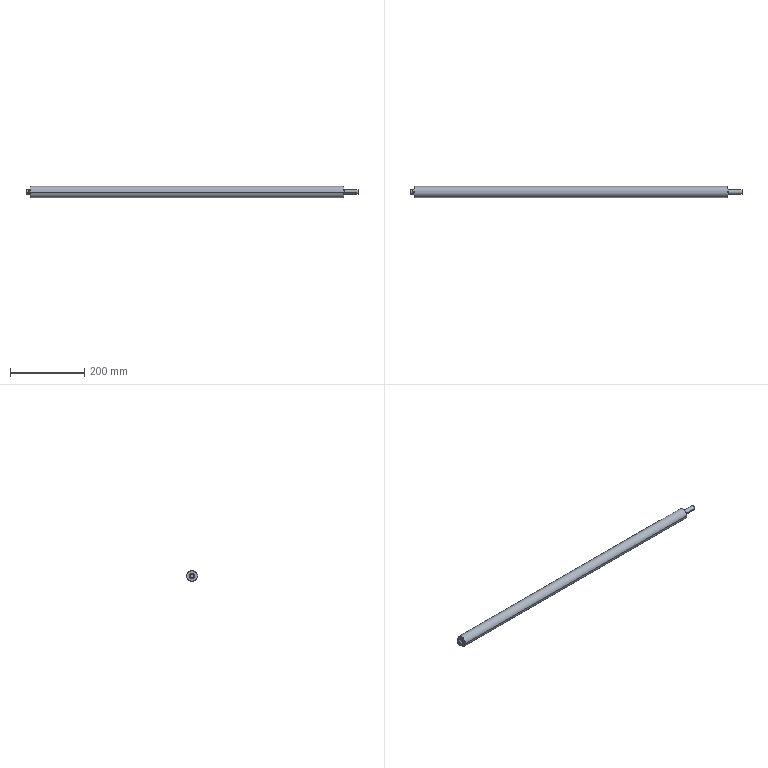Component | SolidWorks | DriveAxis-1_MainFeedAxis3-1 | 1 solid | 26 faces | box 892 x 30 x 30 mm | volume 601650 mm3 | cone 10 | cylinder 10 | plane 6 | commonest cylinder face diameters 12 x4 15 x4 30 x2
build123d program:
from build123d import *

# Parameters (mm, degrees)
SKETCH1_R           = 15
BOSS_EXTRUDE1_DEPTH = 843
SKETCH3_R           = 7.5
BOSS_EXTRUDE2_DEPTH = 3
BOSS_EXTRUDE3_START = 3
SKETCH4_R           = 7.5
BOSS_EXTRUDE3_DEPTH = 3
SKETCH5_R           = 6
BOSS_EXTRUDE4_DEPTH = 35
BOSS_EXTRUDE5_START = 8
SKETCH6_R           = 6
BOSS_EXTRUDE5_DEPTH = 8
CHAMFER1_SIZE       = 1
CHAMFER2_SIZE       = 1


with BuildPart() as part:
    # Sketch1 → Boss-Extrude1 (new body)
    with BuildSketch(Plane.XY):
        with Locations(Location((0, 0, 0), (0, 0, 180))):
            Circle(SKETCH1_R)
    extrude(amount=BOSS_EXTRUDE1_DEPTH)

    # Sketch3 → Boss-Extrude2 (add)
    with BuildSketch(Plane.XY.offset(843)):
        Circle(SKETCH3_R)
    extrude(amount=BOSS_EXTRUDE2_DEPTH)

    # Sketch4 → Boss-Extrude3 (add)
    with BuildSketch(Plane(origin=(0, 0, 0), x_dir=(-1, 0, 0), z_dir=(0, 0, -1)).offset(BOSS_EXTRUDE3_START)):
        with Locations(Location((0, 0, 0), (0, 0, 180))):
            Circle(SKETCH4_R)
    extrude(amount=-BOSS_EXTRUDE3_DEPTH)

    # Sketch5 → Boss-Extrude4 (add)
    with BuildSketch(Plane(origin=(0, 0, -3), x_dir=(-1, 0, 0), z_dir=(0, 0, -1))):
        Circle(SKETCH5_R)
    extrude(amount=BOSS_EXTRUDE4_DEPTH)

    # Sketch6 → Boss-Extrude5 (add)
    with BuildSketch(Plane.XY.offset(846).offset(BOSS_EXTRUDE5_START)):
        with Locations(Location((0, 0, 0), (0, 0, 180))):
            Circle(SKETCH6_R)
    extrude(amount=-BOSS_EXTRUDE5_DEPTH)

    # Chamfer1
    chamfer1_edges = [part.edges().sort_by_distance(p)[0] for p in [
        (6, 0, 854),
        (15, 0, 843),
        (-7.5, 0, 846),
    ]]
    chamfer(chamfer1_edges, length=CHAMFER1_SIZE)

    # Chamfer2
    chamfer2_edges = [part.edges().sort_by_distance(p)[0] for p in [
        (-7.5, 0, -3),
        (15, 0, 0),
    ]]
    chamfer(chamfer2_edges, length=CHAMFER2_SIZE)


solid = part.part

# Placed as in the assembly
solid = solid.moved(Location((856, -30, -142.268), (0, -90, 0)))
STEP:
#1=COLOUR_RGB('',0.7922,0.8196,0.9333);
#2=FILL_AREA_STYLE_COLOUR('',#1);
#3=FILL_AREA_STYLE('',(#2));
#4=SURFACE_STYLE_FILL_AREA(#3);
#5=SURFACE_SIDE_STYLE('',(#4));
#6=SURFACE_STYLE_USAGE(.BOTH.,#5);
#7=PRESENTATION_STYLE_ASSIGNMENT((#6));
#8=CARTESIAN_POINT('',(33.701,-1.732,-5.601));
#9=VERTEX_POINT('',#8);
#10=CARTESIAN_POINT('',(33.701,-0.6299,-5.601));
#11=VERTEX_POINT('',#10);
#12=CARTESIAN_POINT('',(33.701,-1.181,-5.601));
#13=DIRECTION('',(1.,0.,0.));
#14=DIRECTION('',(0.,1.,0.));
#15=AXIS2_PLACEMENT_3D('',#12,#13,#14);
#16=CIRCLE('',#15,0.5512);
#17=EDGE_CURVE('',#9,#11,#16,.T.);
#18=ORIENTED_EDGE('',*,*,#17,.F.);
#19=CARTESIAN_POINT('',(33.661,-1.772,-5.601));
#20=VERTEX_POINT('',#19);
#21=CARTESIAN_POINT('',(33.661,-1.772,-5.601));
#22=DIRECTION('',(-0.7071,-0.7071,-0.));
#23=VECTOR('',#22,39.37);
#24=LINE('',#21,#23);
#25=EDGE_CURVE('',#9,#20,#24,.T.);
#26=ORIENTED_EDGE('',*,*,#25,.T.);
#27=CARTESIAN_POINT('',(33.661,-0.5906,-5.601));
#28=VERTEX_POINT('',#27);
#29=CARTESIAN_POINT('',(33.661,-1.181,-5.601));
#30=DIRECTION('',(-1.,-0.,-0.));
#31=DIRECTION('',(0.,1.,0.));
#32=AXIS2_PLACEMENT_3D('',#29,#30,#31);
#33=CIRCLE('',#32,0.5906);
#34=EDGE_CURVE('',#28,#20,#33,.T.);
#35=ORIENTED_EDGE('',*,*,#34,.F.);
#36=CARTESIAN_POINT('',(33.661,-0.5906,-5.601));
#37=DIRECTION('',(-0.7071,0.7071,0.));
#38=VECTOR('',#37,39.37);
#39=LINE('',#36,#38);
#40=EDGE_CURVE('',#11,#28,#39,.T.);
#41=ORIENTED_EDGE('',*,*,#40,.F.);
#42=EDGE_LOOP('',(#18,#26,#35,#41));
#43=FACE_OUTER_BOUND('',#42,.T.);
#44=CARTESIAN_POINT('',(33.661,-1.181,-5.601));
#45=DIRECTION('',(-1.,-0.,-0.));
#46=DIRECTION('',(0.,1.,0.));
#47=AXIS2_PLACEMENT_3D('',#44,#45,#46);
#48=CONICAL_SURFACE('',#47,0.5906,0.7854);
#49=ADVANCED_FACE('',(#43),#48,.T.);
#50=CARTESIAN_POINT('',(33.819,-1.437,-5.601));
#51=VERTEX_POINT('',#50);
#52=CARTESIAN_POINT('',(33.819,-0.9252,-5.601));
#53=VERTEX_POINT('',#52);
#54=CARTESIAN_POINT('',(33.819,-1.181,-5.601));
#55=DIRECTION('',(1.,0.,0.));
#56=DIRECTION('',(0.,-1.,-0.));
#57=AXIS2_PLACEMENT_3D('',#54,#55,#56);
#58=CIRCLE('',#57,0.2559);
#59=EDGE_CURVE('',#51,#53,#58,.T.);
#60=ORIENTED_EDGE('',*,*,#59,.F.);
#61=CARTESIAN_POINT('',(33.78,-1.476,-5.601));
#62=VERTEX_POINT('',#61);
#63=CARTESIAN_POINT('',(33.819,-1.437,-5.601));
#64=DIRECTION('',(-0.7071,-0.7071,-0.));
#65=VECTOR('',#64,39.37);
#66=LINE('',#63,#65);
#67=EDGE_CURVE('',#51,#62,#66,.T.);
#68=ORIENTED_EDGE('',*,*,#67,.T.);
#69=CARTESIAN_POINT('',(33.78,-0.8858,-5.601));
#70=VERTEX_POINT('',#69);
#71=CARTESIAN_POINT('',(33.78,-1.181,-5.601));
#72=DIRECTION('',(-1.,-0.,-0.));
#73=DIRECTION('',(0.,-1.,-0.));
#74=AXIS2_PLACEMENT_3D('',#71,#72,#73);
#75=CIRCLE('',#74,0.2953);
#76=EDGE_CURVE('',#70,#62,#75,.T.);
#77=ORIENTED_EDGE('',*,*,#76,.F.);
#78=CARTESIAN_POINT('',(33.819,-0.9252,-5.601));
#79=DIRECTION('',(-0.7071,0.7071,0.));
#80=VECTOR('',#79,39.37);
#81=LINE('',#78,#80);
#82=EDGE_CURVE('',#53,#70,#81,.T.);
#83=ORIENTED_EDGE('',*,*,#82,.F.);
#84=EDGE_LOOP('',(#60,#68,#77,#83));
#85=FACE_OUTER_BOUND('',#84,.T.);
#86=CARTESIAN_POINT('',(33.819,-1.181,-5.601));
#87=DIRECTION('',(-1.,-0.,-0.));
#88=DIRECTION('',(0.,1.,0.));
#89=AXIS2_PLACEMENT_3D('',#86,#87,#88);
#90=CONICAL_SURFACE('',#89,0.2559,0.7854);
#91=ADVANCED_FACE('',(#85),#90,.T.);
#92=CARTESIAN_POINT('',(0.5118,-0.6299,-5.601));
#93=VERTEX_POINT('',#92);
#94=CARTESIAN_POINT('',(0.5118,-1.732,-5.601));
#95=VERTEX_POINT('',#94);
#96=CARTESIAN_POINT('',(0.5118,-1.181,-5.601));
#97=DIRECTION('',(-1.,-0.,-0.));
#98=DIRECTION('',(0.,1.,0.));
#99=AXIS2_PLACEMENT_3D('',#96,#97,#98);
#100=CIRCLE('',#99,0.5512);
#101=EDGE_CURVE('',#93,#95,#100,.T.);
#102=ORIENTED_EDGE('',*,*,#101,.F.);
#103=CARTESIAN_POINT('',(0.5512,-0.5906,-5.601));
#104=VERTEX_POINT('',#103);
#105=CARTESIAN_POINT('',(0.5118,-0.6299,-5.601));
#106=DIRECTION('',(0.7071,0.7071,0.));
#107=VECTOR('',#106,39.37);
#108=LINE('',#105,#107);
#109=EDGE_CURVE('',#93,#104,#108,.T.);
#110=ORIENTED_EDGE('',*,*,#109,.T.);
#111=CARTESIAN_POINT('',(0.5512,-1.772,-5.601));
#112=VERTEX_POINT('',#111);
#113=CARTESIAN_POINT('',(0.5512,-1.181,-5.601));
#114=DIRECTION('',(1.,0.,0.));
#115=DIRECTION('',(-0.,1.,0.));
#116=AXIS2_PLACEMENT_3D('',#113,#114,#115);
#117=CIRCLE('',#116,0.5906);
#118=EDGE_CURVE('',#112,#104,#117,.T.);
#119=ORIENTED_EDGE('',*,*,#118,.F.);
#120=CARTESIAN_POINT('',(0.5118,-1.732,-5.601));
#121=DIRECTION('',(0.7071,-0.7071,-0.));
#122=VECTOR('',#121,39.37);
#123=LINE('',#120,#122);
#124=EDGE_CURVE('',#95,#112,#123,.T.);
#125=ORIENTED_EDGE('',*,*,#124,.F.);
#126=EDGE_LOOP('',(#102,#110,#119,#125));
#127=FACE_OUTER_BOUND('',#126,.T.);
#128=CARTESIAN_POINT('',(0.5118,-1.181,-5.601));
#129=DIRECTION('',(1.,0.,0.));
#130=DIRECTION('',(0.,-1.,-0.));
#131=AXIS2_PLACEMENT_3D('',#128,#129,#130);
#132=CONICAL_SURFACE('',#131,0.5512,0.7854);
#133=ADVANCED_FACE('',(#127),#132,.T.);
#134=CARTESIAN_POINT('',(0.3937,-0.9252,-5.601));
#135=VERTEX_POINT('',#134);
#136=CARTESIAN_POINT('',(0.3937,-1.437,-5.601));
#137=VERTEX_POINT('',#136);
#138=CARTESIAN_POINT('',(0.3937,-1.181,-5.601));
#139=DIRECTION('',(-1.,-0.,-0.));
#140=DIRECTION('',(0.,1.,0.));
#141=AXIS2_PLACEMENT_3D('',#138,#139,#140);
#142=CIRCLE('',#141,0.2559);
#143=EDGE_CURVE('',#135,#137,#142,.T.);
#144=ORIENTED_EDGE('',*,*,#143,.F.);
#145=CARTESIAN_POINT('',(0.4331,-0.8858,-5.601));
#146=VERTEX_POINT('',#145);
#147=CARTESIAN_POINT('',(0.3937,-0.9252,-5.601));
#148=DIRECTION('',(0.7071,0.7071,0.));
#149=VECTOR('',#148,39.37);
#150=LINE('',#147,#149);
#151=EDGE_CURVE('',#135,#146,#150,.T.);
#152=ORIENTED_EDGE('',*,*,#151,.T.);
#153=CARTESIAN_POINT('',(0.4331,-1.476,-5.601));
#154=VERTEX_POINT('',#153);
#155=CARTESIAN_POINT('',(0.4331,-1.181,-5.601));
#156=DIRECTION('',(1.,0.,0.));
#157=DIRECTION('',(0.,1.,0.));
#158=AXIS2_PLACEMENT_3D('',#155,#156,#157);
#159=CIRCLE('',#158,0.2953);
#160=EDGE_CURVE('',#154,#146,#159,.T.);
#161=ORIENTED_EDGE('',*,*,#160,.F.);
#162=CARTESIAN_POINT('',(0.3937,-1.437,-5.601));
#163=DIRECTION('',(0.7071,-0.7071,-0.));
#164=VECTOR('',#163,39.37);
#165=LINE('',#162,#164);
#166=EDGE_CURVE('',#137,#154,#165,.T.);
#167=ORIENTED_EDGE('',*,*,#166,.F.);
#168=EDGE_LOOP('',(#144,#152,#161,#167));
#169=FACE_OUTER_BOUND('',#168,.T.);
#170=CARTESIAN_POINT('',(0.3937,-1.181,-5.601));
#171=DIRECTION('',(1.,0.,0.));
#172=DIRECTION('',(0.,-1.,-0.));
#173=AXIS2_PLACEMENT_3D('',#170,#171,#172);
#174=CONICAL_SURFACE('',#173,0.2559,0.7854);
#175=ADVANCED_FACE('',(#169),#174,.T.);
#176=CARTESIAN_POINT('',(0.07874,-0.9843,-5.601));
#177=VERTEX_POINT('',#176);
#178=CARTESIAN_POINT('',(0.07874,-1.378,-5.601));
#179=VERTEX_POINT('',#178);
#180=CARTESIAN_POINT('',(0.07874,-1.181,-5.601));
#181=DIRECTION('',(-1.,-0.,-0.));
#182=DIRECTION('',(-0.,1.,0.));
#183=AXIS2_PLACEMENT_3D('',#180,#181,#182);
#184=CIRCLE('',#183,0.1969);
#185=EDGE_CURVE('',#177,#179,#184,.T.);
#186=ORIENTED_EDGE('',*,*,#185,.F.);
#187=CARTESIAN_POINT('',(0.1181,-0.9449,-5.601));
#188=VERTEX_POINT('',#187);
#189=CARTESIAN_POINT('',(0.07874,-0.9843,-5.601));
#190=DIRECTION('',(0.7071,0.7071,0.));
#191=VECTOR('',#190,39.37);
#192=LINE('',#189,#191);
#193=EDGE_CURVE('',#177,#188,#192,.T.);
#194=ORIENTED_EDGE('',*,*,#193,.T.);
#195=CARTESIAN_POINT('',(0.1181,-1.417,-5.601));
#196=VERTEX_POINT('',#195);
#197=CARTESIAN_POINT('',(0.1181,-1.181,-5.601));
#198=DIRECTION('',(1.,0.,0.));
#199=DIRECTION('',(-0.,1.,0.));
#200=AXIS2_PLACEMENT_3D('',#197,#198,#199);
#201=CIRCLE('',#200,0.2362);
#202=EDGE_CURVE('',#196,#188,#201,.T.);
#203=ORIENTED_EDGE('',*,*,#202,.F.);
#204=CARTESIAN_POINT('',(0.07874,-1.378,-5.601));
#205=DIRECTION('',(0.7071,-0.7071,-0.));
#206=VECTOR('',#205,39.37);
#207=LINE('',#204,#206);
#208=EDGE_CURVE('',#179,#196,#207,.T.);
#209=ORIENTED_EDGE('',*,*,#208,.F.);
#210=EDGE_LOOP('',(#186,#194,#203,#209));
#211=FACE_OUTER_BOUND('',#210,.T.);
#212=CARTESIAN_POINT('',(0.07874,-1.181,-5.601));
#213=DIRECTION('',(1.,0.,0.));
#214=DIRECTION('',(0.,-1.,-0.));
#215=AXIS2_PLACEMENT_3D('',#212,#213,#214);
#216=CONICAL_SURFACE('',#215,0.1969,0.7854);
#217=ADVANCED_FACE('',(#211),#216,.T.);
#218=ORIENTED_EDGE('',*,*,#202,.T.);
#219=CARTESIAN_POINT('',(0.3937,-0.9449,-5.601));
#220=VERTEX_POINT('',#219);
#221=CARTESIAN_POINT('',(0.07874,-0.9449,-5.601));
#222=DIRECTION('',(1.,0.,0.));
#223=VECTOR('',#222,39.37);
#224=LINE('',#221,#223);
#225=EDGE_CURVE('',#188,#220,#224,.T.);
#226=ORIENTED_EDGE('',*,*,#225,.T.);
#227=CARTESIAN_POINT('',(0.3937,-1.417,-5.601));
#228=VERTEX_POINT('',#227);
#229=CARTESIAN_POINT('',(0.3937,-1.181,-5.601));
#230=DIRECTION('',(-1.,-0.,-0.));
#231=DIRECTION('',(0.,1.,0.));
#232=AXIS2_PLACEMENT_3D('',#229,#230,#231);
#233=CIRCLE('',#232,0.2362);
#234=EDGE_CURVE('',#220,#228,#233,.T.);
#235=ORIENTED_EDGE('',*,*,#234,.T.);
#236=CARTESIAN_POINT('',(0.07874,-1.417,-5.601));
#237=DIRECTION('',(1.,0.,0.));
#238=VECTOR('',#237,39.37);
#239=LINE('',#236,#238);
#240=EDGE_CURVE('',#196,#228,#239,.T.);
#241=ORIENTED_EDGE('',*,*,#240,.F.);
#242=EDGE_LOOP('',(#218,#226,#235,#241));
#243=FACE_OUTER_BOUND('',#242,.T.);
#244=CARTESIAN_POINT('',(0.07874,-1.181,-5.601));
#245=DIRECTION('',(1.,0.,0.));
#246=DIRECTION('',(0.,-1.,-0.));
#247=AXIS2_PLACEMENT_3D('',#244,#245,#246);
#248=CYLINDRICAL_SURFACE('',#247,0.2362);
#249=ADVANCED_FACE('',(#243),#248,.T.);
#250=CARTESIAN_POINT('',(35.197,-1.417,-5.601));
#251=VERTEX_POINT('',#250);
#252=CARTESIAN_POINT('',(35.197,-0.9449,-5.601));
#253=VERTEX_POINT('',#252);
#254=CARTESIAN_POINT('',(35.197,-1.181,-5.601));
#255=DIRECTION('',(1.,0.,0.));
#256=DIRECTION('',(0.,-1.,-0.));
#257=AXIS2_PLACEMENT_3D('',#254,#255,#256);
#258=CIRCLE('',#257,0.2362);
#259=EDGE_CURVE('',#251,#253,#258,.T.);
#260=ORIENTED_EDGE('',*,*,#259,.F.);
#261=CARTESIAN_POINT('',(33.819,-1.417,-5.601));
#262=VERTEX_POINT('',#261);
#263=CARTESIAN_POINT('',(35.197,-1.417,-5.601));
#264=DIRECTION('',(-1.,-0.,-0.));
#265=VECTOR('',#264,39.37);
#266=LINE('',#263,#265);
#267=EDGE_CURVE('',#251,#262,#266,.T.);
#268=ORIENTED_EDGE('',*,*,#267,.T.);
#269=CARTESIAN_POINT('',(33.819,-0.9449,-5.601));
#270=VERTEX_POINT('',#269);
#271=CARTESIAN_POINT('',(33.819,-1.181,-5.601));
#272=DIRECTION('',(1.,0.,0.));
#273=DIRECTION('',(0.,-1.,-0.));
#274=AXIS2_PLACEMENT_3D('',#271,#272,#273);
#275=CIRCLE('',#274,0.2362);
#276=EDGE_CURVE('',#262,#270,#275,.T.);
#277=ORIENTED_EDGE('',*,*,#276,.T.);
#278=CARTESIAN_POINT('',(35.197,-0.9449,-5.601));
#279=DIRECTION('',(-1.,-0.,-0.));
#280=VECTOR('',#279,39.37);
#281=LINE('',#278,#280);
#282=EDGE_CURVE('',#253,#270,#281,.T.);
#283=ORIENTED_EDGE('',*,*,#282,.F.);
#284=EDGE_LOOP('',(#260,#268,#277,#283));
#285=FACE_OUTER_BOUND('',#284,.T.);
#286=CARTESIAN_POINT('',(35.197,-1.181,-5.601));
#287=DIRECTION('',(-1.,-0.,-0.));
#288=DIRECTION('',(0.,1.,0.));
#289=AXIS2_PLACEMENT_3D('',#286,#287,#288);
#290=CYLINDRICAL_SURFACE('',#289,0.2362);
#291=ADVANCED_FACE('',(#285),#290,.T.);
#292=ORIENTED_EDGE('',*,*,#76,.T.);
#293=CARTESIAN_POINT('',(33.701,-1.476,-5.601));
#294=VERTEX_POINT('',#293);
#295=CARTESIAN_POINT('',(33.819,-1.476,-5.601));
#296=DIRECTION('',(-1.,-0.,-0.));
#297=VECTOR('',#296,39.37);
#298=LINE('',#295,#297);
#299=EDGE_CURVE('',#62,#294,#298,.T.);
#300=ORIENTED_EDGE('',*,*,#299,.T.);
#301=CARTESIAN_POINT('',(33.701,-0.8858,-5.601));
#302=VERTEX_POINT('',#301);
#303=CARTESIAN_POINT('',(33.701,-1.181,-5.601));
#304=DIRECTION('',(1.,0.,0.));
#305=DIRECTION('',(0.,1.,0.));
#306=AXIS2_PLACEMENT_3D('',#303,#304,#305);
#307=CIRCLE('',#306,0.2953);
#308=EDGE_CURVE('',#294,#302,#307,.T.);
#309=ORIENTED_EDGE('',*,*,#308,.T.);
#310=CARTESIAN_POINT('',(33.819,-0.8858,-5.601));
#311=DIRECTION('',(-1.,-0.,-0.));
#312=VECTOR('',#311,39.37);
#313=LINE('',#310,#312);
#314=EDGE_CURVE('',#70,#302,#313,.T.);
#315=ORIENTED_EDGE('',*,*,#314,.F.);
#316=EDGE_LOOP('',(#292,#300,#309,#315));
#317=FACE_OUTER_BOUND('',#316,.T.);
#318=CARTESIAN_POINT('',(33.819,-1.181,-5.601));
#319=DIRECTION('',(-1.,-0.,-0.));
#320=DIRECTION('',(0.,1.,0.));
#321=AXIS2_PLACEMENT_3D('',#318,#319,#320);
#322=CYLINDRICAL_SURFACE('',#321,0.2953);
#323=ADVANCED_FACE('',(#317),#322,.T.);
#324=ORIENTED_EDGE('',*,*,#160,.T.);
#325=CARTESIAN_POINT('',(0.5118,-0.8858,-5.601));
#326=VERTEX_POINT('',#325);
#327=CARTESIAN_POINT('',(0.3937,-0.8858,-5.601));
#328=DIRECTION('',(1.,0.,0.));
#329=VECTOR('',#328,39.37);
#330=LINE('',#327,#329);
#331=EDGE_CURVE('',#146,#326,#330,.T.);
#332=ORIENTED_EDGE('',*,*,#331,.T.);
#333=CARTESIAN_POINT('',(0.5118,-1.476,-5.601));
#334=VERTEX_POINT('',#333);
#335=CARTESIAN_POINT('',(0.5118,-1.181,-5.601));
#336=DIRECTION('',(-1.,-0.,-0.));
#337=DIRECTION('',(0.,1.,0.));
#338=AXIS2_PLACEMENT_3D('',#335,#336,#337);
#339=CIRCLE('',#338,0.2953);
#340=EDGE_CURVE('',#326,#334,#339,.T.);
#341=ORIENTED_EDGE('',*,*,#340,.T.);
#342=CARTESIAN_POINT('',(0.3937,-1.476,-5.601));
#343=DIRECTION('',(1.,0.,0.));
#344=VECTOR('',#343,39.37);
#345=LINE('',#342,#344);
#346=EDGE_CURVE('',#154,#334,#345,.T.);
#347=ORIENTED_EDGE('',*,*,#346,.F.);
#348=EDGE_LOOP('',(#324,#332,#341,#347));
#349=FACE_OUTER_BOUND('',#348,.T.);
#350=CARTESIAN_POINT('',(0.3937,-1.181,-5.601));
#351=DIRECTION('',(1.,0.,0.));
#352=DIRECTION('',(0.,-1.,-0.));
#353=AXIS2_PLACEMENT_3D('',#350,#351,#352);
#354=CYLINDRICAL_SURFACE('',#353,0.2953);
#355=ADVANCED_FACE('',(#349),#354,.T.);
#356=ORIENTED_EDGE('',*,*,#118,.T.);
#357=CARTESIAN_POINT('',(0.5118,-0.5906,-5.601));
#358=DIRECTION('',(1.,0.,0.));
#359=VECTOR('',#358,39.37);
#360=LINE('',#357,#359);
#361=EDGE_CURVE('',#104,#28,#360,.T.);
#362=ORIENTED_EDGE('',*,*,#361,.T.);
#363=ORIENTED_EDGE('',*,*,#34,.T.);
#364=CARTESIAN_POINT('',(0.5118,-1.772,-5.601));
#365=DIRECTION('',(1.,0.,0.));
#366=VECTOR('',#365,39.37);
#367=LINE('',#364,#366);
#368=EDGE_CURVE('',#112,#20,#367,.T.);
#369=ORIENTED_EDGE('',*,*,#368,.F.);
#370=EDGE_LOOP('',(#356,#362,#363,#369));
#371=FACE_OUTER_BOUND('',#370,.T.);
#372=CARTESIAN_POINT('',(0.5118,-1.181,-5.601));
#373=DIRECTION('',(1.,0.,0.));
#374=DIRECTION('',(0.,-1.,-0.));
#375=AXIS2_PLACEMENT_3D('',#372,#373,#374);
#376=CYLINDRICAL_SURFACE('',#375,0.5906);
#377=ADVANCED_FACE('',(#371),#376,.T.);
#378=ORIENTED_EDGE('',*,*,#361,.F.);
#379=CARTESIAN_POINT('',(0.5512,-1.181,-5.601));
#380=DIRECTION('',(1.,0.,0.));
#381=DIRECTION('',(-0.,1.,0.));
#382=AXIS2_PLACEMENT_3D('',#379,#380,#381);
#383=CIRCLE('',#382,0.5906);
#384=EDGE_CURVE('',#104,#112,#383,.T.);
#385=ORIENTED_EDGE('',*,*,#384,.T.);
#386=ORIENTED_EDGE('',*,*,#368,.T.);
#387=CARTESIAN_POINT('',(33.661,-1.181,-5.601));
#388=DIRECTION('',(-1.,-0.,-0.));
#389=DIRECTION('',(0.,1.,0.));
#390=AXIS2_PLACEMENT_3D('',#387,#388,#389);
#391=CIRCLE('',#390,0.5906);
#392=EDGE_CURVE('',#20,#28,#391,.T.);
#393=ORIENTED_EDGE('',*,*,#392,.T.);
#394=EDGE_LOOP('',(#378,#385,#386,#393));
#395=FACE_OUTER_BOUND('',#394,.T.);
#396=CARTESIAN_POINT('',(0.5118,-1.181,-5.601));
#397=DIRECTION('',(1.,0.,0.));
#398=DIRECTION('',(0.,-1.,-0.));
#399=AXIS2_PLACEMENT_3D('',#396,#397,#398);
#400=CYLINDRICAL_SURFACE('',#399,0.5906);
#401=ADVANCED_FACE('',(#395),#400,.T.);
#402=CARTESIAN_POINT('',(0.5118,-1.181,-5.601));
#403=DIRECTION('',(-1.,-0.,-0.));
#404=DIRECTION('',(0.,1.,0.));
#405=AXIS2_PLACEMENT_3D('',#402,#403,#404);
#406=CIRCLE('',#405,0.5512);
#407=EDGE_CURVE('',#95,#93,#406,.T.);
#408=ORIENTED_EDGE('',*,*,#407,.T.);
#409=ORIENTED_EDGE('',*,*,#101,.T.);
#410=EDGE_LOOP('',(#408,#409));
#411=FACE_OUTER_BOUND('',#410,.T.);
#412=CARTESIAN_POINT('',(0.5118,-1.181,-5.601));
#413=DIRECTION('',(-1.,-0.,-0.));
#414=DIRECTION('',(0.,1.,0.));
#415=AXIS2_PLACEMENT_3D('',#412,#413,#414);
#416=CIRCLE('',#415,0.2953);
#417=EDGE_CURVE('',#334,#326,#416,.T.);
#418=ORIENTED_EDGE('',*,*,#417,.F.);
#419=ORIENTED_EDGE('',*,*,#340,.F.);
#420=EDGE_LOOP('',(#418,#419));
#421=FACE_BOUND('',#420,.T.);
#422=CARTESIAN_POINT('',(0.5118,-1.181,-5.601));
#423=DIRECTION('',(-1.,-0.,-0.));
#424=DIRECTION('',(-0.,1.,0.));
#425=AXIS2_PLACEMENT_3D('',#422,#423,#424);
#426=PLANE('',#425);
#427=ADVANCED_FACE('',(#411,#421),#426,.T.);
#428=CARTESIAN_POINT('',(33.701,-1.181,-5.601));
#429=DIRECTION('',(1.,0.,0.));
#430=DIRECTION('',(0.,1.,0.));
#431=AXIS2_PLACEMENT_3D('',#428,#429,#430);
#432=CIRCLE('',#431,0.5512);
#433=EDGE_CURVE('',#11,#9,#432,.T.);
#434=ORIENTED_EDGE('',*,*,#433,.T.);
#435=ORIENTED_EDGE('',*,*,#17,.T.);
#436=EDGE_LOOP('',(#434,#435));
#437=FACE_OUTER_BOUND('',#436,.T.);
#438=CARTESIAN_POINT('',(33.701,-1.181,-5.601));
#439=DIRECTION('',(1.,0.,0.));
#440=DIRECTION('',(0.,1.,0.));
#441=AXIS2_PLACEMENT_3D('',#438,#439,#440);
#442=CIRCLE('',#441,0.2953);
#443=EDGE_CURVE('',#302,#294,#442,.T.);
#444=ORIENTED_EDGE('',*,*,#443,.F.);
#445=ORIENTED_EDGE('',*,*,#308,.F.);
#446=EDGE_LOOP('',(#444,#445));
#447=FACE_BOUND('',#446,.T.);
#448=CARTESIAN_POINT('',(33.701,-1.181,-5.601));
#449=DIRECTION('',(-1.,-0.,-0.));
#450=DIRECTION('',(-0.,1.,0.));
#451=AXIS2_PLACEMENT_3D('',#448,#449,#450);
#452=PLANE('',#451);
#453=ADVANCED_FACE('',(#437,#447),#452,.F.);
#454=ORIENTED_EDGE('',*,*,#331,.F.);
#455=CARTESIAN_POINT('',(0.4331,-1.181,-5.601));
#456=DIRECTION('',(1.,0.,0.));
#457=DIRECTION('',(0.,1.,0.));
#458=AXIS2_PLACEMENT_3D('',#455,#456,#457);
#459=CIRCLE('',#458,0.2953);
#460=EDGE_CURVE('',#146,#154,#459,.T.);
#461=ORIENTED_EDGE('',*,*,#460,.T.);
#462=ORIENTED_EDGE('',*,*,#346,.T.);
#463=ORIENTED_EDGE('',*,*,#417,.T.);
#464=EDGE_LOOP('',(#454,#461,#462,#463));
#465=FACE_OUTER_BOUND('',#464,.T.);
#466=CARTESIAN_POINT('',(0.3937,-1.181,-5.601));
#467=DIRECTION('',(1.,0.,0.));
#468=DIRECTION('',(0.,-1.,-0.));
#469=AXIS2_PLACEMENT_3D('',#466,#467,#468);
#470=CYLINDRICAL_SURFACE('',#469,0.2953);
#471=ADVANCED_FACE('',(#465),#470,.T.);
#472=CARTESIAN_POINT('',(0.3937,-1.181,-5.601));
#473=DIRECTION('',(-1.,-0.,-0.));
#474=DIRECTION('',(0.,1.,0.));
#475=AXIS2_PLACEMENT_3D('',#472,#473,#474);
#476=CIRCLE('',#475,0.2559);
#477=EDGE_CURVE('',#137,#135,#476,.T.);
#478=ORIENTED_EDGE('',*,*,#477,.T.);
#479=ORIENTED_EDGE('',*,*,#143,.T.);
#480=EDGE_LOOP('',(#478,#479));
#481=FACE_OUTER_BOUND('',#480,.T.);
#482=CARTESIAN_POINT('',(0.3937,-1.181,-5.601));
#483=DIRECTION('',(-1.,-0.,-0.));
#484=DIRECTION('',(0.,1.,0.));
#485=AXIS2_PLACEMENT_3D('',#482,#483,#484);
#486=CIRCLE('',#485,0.2362);
#487=EDGE_CURVE('',#228,#220,#486,.T.);
#488=ORIENTED_EDGE('',*,*,#487,.F.);
#489=ORIENTED_EDGE('',*,*,#234,.F.);
#490=EDGE_LOOP('',(#488,#489));
#491=FACE_BOUND('',#490,.T.);
#492=CARTESIAN_POINT('',(0.3937,-1.181,-5.601));
#493=DIRECTION('',(-1.,-0.,-0.));
#494=DIRECTION('',(-0.,1.,0.));
#495=AXIS2_PLACEMENT_3D('',#492,#493,#494);
#496=PLANE('',#495);
#497=ADVANCED_FACE('',(#481,#491),#496,.T.);
#498=ORIENTED_EDGE('',*,*,#299,.F.);
#499=CARTESIAN_POINT('',(33.78,-1.181,-5.601));
#500=DIRECTION('',(-1.,-0.,-0.));
#501=DIRECTION('',(0.,-1.,-0.));
#502=AXIS2_PLACEMENT_3D('',#499,#500,#501);
#503=CIRCLE('',#502,0.2953);
#504=EDGE_CURVE('',#62,#70,#503,.T.);
#505=ORIENTED_EDGE('',*,*,#504,.T.);
#506=ORIENTED_EDGE('',*,*,#314,.T.);
#507=ORIENTED_EDGE('',*,*,#443,.T.);
#508=EDGE_LOOP('',(#498,#505,#506,#507));
#509=FACE_OUTER_BOUND('',#508,.T.);
#510=CARTESIAN_POINT('',(33.819,-1.181,-5.601));
#511=DIRECTION('',(-1.,-0.,-0.));
#512=DIRECTION('',(0.,1.,0.));
#513=AXIS2_PLACEMENT_3D('',#510,#511,#512);
#514=CYLINDRICAL_SURFACE('',#513,0.2953);
#515=ADVANCED_FACE('',(#509),#514,.T.);
#516=CARTESIAN_POINT('',(33.819,-1.181,-5.601));
#517=DIRECTION('',(1.,0.,0.));
#518=DIRECTION('',(0.,-1.,-0.));
#519=AXIS2_PLACEMENT_3D('',#516,#517,#518);
#520=CIRCLE('',#519,0.2559);
#521=EDGE_CURVE('',#53,#51,#520,.T.);
#522=ORIENTED_EDGE('',*,*,#521,.T.);
#523=ORIENTED_EDGE('',*,*,#59,.T.);
#524=EDGE_LOOP('',(#522,#523));
#525=FACE_OUTER_BOUND('',#524,.T.);
#526=CARTESIAN_POINT('',(33.819,-1.181,-5.601));
#527=DIRECTION('',(1.,0.,0.));
#528=DIRECTION('',(0.,-1.,-0.));
#529=AXIS2_PLACEMENT_3D('',#526,#527,#528);
#530=CIRCLE('',#529,0.2362);
#531=EDGE_CURVE('',#270,#262,#530,.T.);
#532=ORIENTED_EDGE('',*,*,#531,.F.);
#533=ORIENTED_EDGE('',*,*,#276,.F.);
#534=EDGE_LOOP('',(#532,#533));
#535=FACE_BOUND('',#534,.T.);
#536=CARTESIAN_POINT('',(33.819,-1.181,-5.601));
#537=DIRECTION('',(1.,0.,0.));
#538=DIRECTION('',(0.,-1.,-0.));
#539=AXIS2_PLACEMENT_3D('',#536,#537,#538);
#540=PLANE('',#539);
#541=ADVANCED_FACE('',(#525,#535),#540,.T.);
#542=ORIENTED_EDGE('',*,*,#267,.F.);
#543=CARTESIAN_POINT('',(35.197,-1.181,-5.601));
#544=DIRECTION('',(1.,0.,0.));
#545=DIRECTION('',(0.,-1.,-0.));
#546=AXIS2_PLACEMENT_3D('',#543,#544,#545);
#547=CIRCLE('',#546,0.2362);
#548=EDGE_CURVE('',#253,#251,#547,.T.);
#549=ORIENTED_EDGE('',*,*,#548,.F.);
#550=ORIENTED_EDGE('',*,*,#282,.T.);
#551=ORIENTED_EDGE('',*,*,#531,.T.);
#552=EDGE_LOOP('',(#542,#549,#550,#551));
#553=FACE_OUTER_BOUND('',#552,.T.);
#554=CARTESIAN_POINT('',(35.197,-1.181,-5.601));
#555=DIRECTION('',(-1.,-0.,-0.));
#556=DIRECTION('',(0.,1.,0.));
#557=AXIS2_PLACEMENT_3D('',#554,#555,#556);
#558=CYLINDRICAL_SURFACE('',#557,0.2362);
#559=ADVANCED_FACE('',(#553),#558,.T.);
#560=ORIENTED_EDGE('',*,*,#548,.T.);
#561=ORIENTED_EDGE('',*,*,#259,.T.);
#562=EDGE_LOOP('',(#560,#561));
#563=FACE_OUTER_BOUND('',#562,.T.);
#564=CARTESIAN_POINT('',(35.197,-1.181,-5.601));
#565=DIRECTION('',(1.,0.,0.));
#566=DIRECTION('',(0.,-1.,-0.));
#567=AXIS2_PLACEMENT_3D('',#564,#565,#566);
#568=PLANE('',#567);
#569=ADVANCED_FACE('',(#563),#568,.T.);
#570=ORIENTED_EDGE('',*,*,#225,.F.);
#571=CARTESIAN_POINT('',(0.1181,-1.181,-5.601));
#572=DIRECTION('',(1.,0.,0.));
#573=DIRECTION('',(-0.,1.,0.));
#574=AXIS2_PLACEMENT_3D('',#571,#572,#573);
#575=CIRCLE('',#574,0.2362);
#576=EDGE_CURVE('',#188,#196,#575,.T.);
#577=ORIENTED_EDGE('',*,*,#576,.T.);
#578=ORIENTED_EDGE('',*,*,#240,.T.);
#579=ORIENTED_EDGE('',*,*,#487,.T.);
#580=EDGE_LOOP('',(#570,#577,#578,#579));
#581=FACE_OUTER_BOUND('',#580,.T.);
#582=CARTESIAN_POINT('',(0.07874,-1.181,-5.601));
#583=DIRECTION('',(1.,0.,0.));
#584=DIRECTION('',(0.,-1.,-0.));
#585=AXIS2_PLACEMENT_3D('',#582,#583,#584);
#586=CYLINDRICAL_SURFACE('',#585,0.2362);
#587=ADVANCED_FACE('',(#581),#586,.T.);
#588=CARTESIAN_POINT('',(0.07874,-1.181,-5.601));
#589=DIRECTION('',(-1.,-0.,-0.));
#590=DIRECTION('',(-0.,1.,0.));
#591=AXIS2_PLACEMENT_3D('',#588,#589,#590);
#592=CIRCLE('',#591,0.1969);
#593=EDGE_CURVE('',#179,#177,#592,.T.);
#594=ORIENTED_EDGE('',*,*,#593,.T.);
#595=ORIENTED_EDGE('',*,*,#185,.T.);
#596=EDGE_LOOP('',(#594,#595));
#597=FACE_OUTER_BOUND('',#596,.T.);
#598=CARTESIAN_POINT('',(0.07874,-1.181,-5.601));
#599=DIRECTION('',(-1.,-0.,-0.));
#600=DIRECTION('',(-0.,1.,0.));
#601=AXIS2_PLACEMENT_3D('',#598,#599,#600);
#602=PLANE('',#601);
#603=ADVANCED_FACE('',(#597),#602,.T.);
#604=ORIENTED_EDGE('',*,*,#193,.F.);
#605=ORIENTED_EDGE('',*,*,#593,.F.);
#606=ORIENTED_EDGE('',*,*,#208,.T.);
#607=ORIENTED_EDGE('',*,*,#576,.F.);
#608=EDGE_LOOP('',(#604,#605,#606,#607));
#609=FACE_OUTER_BOUND('',#608,.T.);
#610=CARTESIAN_POINT('',(0.07874,-1.181,-5.601));
#611=DIRECTION('',(1.,0.,0.));
#612=DIRECTION('',(0.,-1.,-0.));
#613=AXIS2_PLACEMENT_3D('',#610,#611,#612);
#614=CONICAL_SURFACE('',#613,0.1969,0.7854);
#615=ADVANCED_FACE('',(#609),#614,.T.);
#616=ORIENTED_EDGE('',*,*,#151,.F.);
#617=ORIENTED_EDGE('',*,*,#477,.F.);
#618=ORIENTED_EDGE('',*,*,#166,.T.);
#619=ORIENTED_EDGE('',*,*,#460,.F.);
#620=EDGE_LOOP('',(#616,#617,#618,#619));
#621=FACE_OUTER_BOUND('',#620,.T.);
#622=CARTESIAN_POINT('',(0.3937,-1.181,-5.601));
#623=DIRECTION('',(1.,0.,0.));
#624=DIRECTION('',(0.,-1.,-0.));
#625=AXIS2_PLACEMENT_3D('',#622,#623,#624);
#626=CONICAL_SURFACE('',#625,0.2559,0.7854);
#627=ADVANCED_FACE('',(#621),#626,.T.);
#628=ORIENTED_EDGE('',*,*,#109,.F.);
#629=ORIENTED_EDGE('',*,*,#407,.F.);
#630=ORIENTED_EDGE('',*,*,#124,.T.);
#631=ORIENTED_EDGE('',*,*,#384,.F.);
#632=EDGE_LOOP('',(#628,#629,#630,#631));
#633=FACE_OUTER_BOUND('',#632,.T.);
#634=CARTESIAN_POINT('',(0.5118,-1.181,-5.601));
#635=DIRECTION('',(1.,0.,0.));
#636=DIRECTION('',(0.,-1.,-0.));
#637=AXIS2_PLACEMENT_3D('',#634,#635,#636);
#638=CONICAL_SURFACE('',#637,0.5512,0.7854);
#639=ADVANCED_FACE('',(#633),#638,.T.);
#640=ORIENTED_EDGE('',*,*,#67,.F.);
#641=ORIENTED_EDGE('',*,*,#521,.F.);
#642=ORIENTED_EDGE('',*,*,#82,.T.);
#643=ORIENTED_EDGE('',*,*,#504,.F.);
#644=EDGE_LOOP('',(#640,#641,#642,#643));
#645=FACE_OUTER_BOUND('',#644,.T.);
#646=CARTESIAN_POINT('',(33.819,-1.181,-5.601));
#647=DIRECTION('',(-1.,-0.,-0.));
#648=DIRECTION('',(0.,1.,0.));
#649=AXIS2_PLACEMENT_3D('',#646,#647,#648);
#650=CONICAL_SURFACE('',#649,0.2559,0.7854);
#651=ADVANCED_FACE('',(#645),#650,.T.);
#652=ORIENTED_EDGE('',*,*,#25,.F.);
#653=ORIENTED_EDGE('',*,*,#433,.F.);
#654=ORIENTED_EDGE('',*,*,#40,.T.);
#655=ORIENTED_EDGE('',*,*,#392,.F.);
#656=EDGE_LOOP('',(#652,#653,#654,#655));
#657=FACE_OUTER_BOUND('',#656,.T.);
#658=CARTESIAN_POINT('',(33.661,-1.181,-5.601));
#659=DIRECTION('',(-1.,-0.,-0.));
#660=DIRECTION('',(0.,1.,0.));
#661=AXIS2_PLACEMENT_3D('',#658,#659,#660);
#662=CONICAL_SURFACE('',#661,0.5906,0.7854);
#663=ADVANCED_FACE('',(#657),#662,.T.);
#664=CLOSED_SHELL('',(#49,#91,#133,#175,#217,#249,#291,#323,#355,#377,#401,#427,#453,#471,#497,#515,#541,#559,#569,#587,#603,#615,#627,#639,#651,#663));
#665=MANIFOLD_SOLID_BREP('',#664);
#666=STYLED_ITEM('',(#7),#665);
#667=PRESENTATION_LAYER_ASSIGNMENT('','',(#666));
#668=CARTESIAN_POINT('',(0.,0.,0.));
#669=DIRECTION('',(0.,0.,1.));
#670=DIRECTION('',(1.,0.,0.));
#671=AXIS2_PLACEMENT_3D('',#668,#669,#670);
#672=(LENGTH_UNIT()NAMED_UNIT(*)SI_UNIT($,.METRE.));
#673=LENGTH_MEASURE_WITH_UNIT(LENGTH_MEASURE(0.0254),#672);
#674=DIMENSIONAL_EXPONENTS(1.,0.,0.,0.,0.,0.,0.);
#675=(CONVERSION_BASED_UNIT('',#673)LENGTH_UNIT()NAMED_UNIT(#674));
#676=UNCERTAINTY_MEASURE_WITH_UNIT(LENGTH_MEASURE(0.00001),#675,'','');
#677=(NAMED_UNIT(*)PLANE_ANGLE_UNIT()SI_UNIT($,.RADIAN.));
#678=(NAMED_UNIT(*)SI_UNIT($,.STERADIAN.)SOLID_ANGLE_UNIT());
#679=(GEOMETRIC_REPRESENTATION_CONTEXT(3)GLOBAL_UNCERTAINTY_ASSIGNED_CONTEXT((#676))GLOBAL_UNIT_ASSIGNED_CONTEXT((#675,#677,#678))REPRESENTATION_CONTEXT('',''));
#680=ADVANCED_BREP_SHAPE_REPRESENTATION('',(#665,#671),#679);
#681=(LENGTH_UNIT()NAMED_UNIT(*)SI_UNIT($,.METRE.));
#682=LENGTH_MEASURE_WITH_UNIT(LENGTH_MEASURE(0.0254),#681);
#683=DIMENSIONAL_EXPONENTS(1.,0.,0.,0.,0.,0.,0.);
#684=(CONVERSION_BASED_UNIT('',#682)LENGTH_UNIT()NAMED_UNIT(#683));
#685=UNCERTAINTY_MEASURE_WITH_UNIT(LENGTH_MEASURE(0.00001),#684,'','');
#686=(NAMED_UNIT(*)PLANE_ANGLE_UNIT()SI_UNIT($,.RADIAN.));
#687=(NAMED_UNIT(*)SI_UNIT($,.STERADIAN.)SOLID_ANGLE_UNIT());
#688=(GEOMETRIC_REPRESENTATION_CONTEXT(3)GLOBAL_UNCERTAINTY_ASSIGNED_CONTEXT((#685))GLOBAL_UNIT_ASSIGNED_CONTEXT((#684,#686,#687))REPRESENTATION_CONTEXT('',''));
#689=MECHANICAL_DESIGN_GEOMETRIC_PRESENTATION_REPRESENTATION('',(#666),#688);